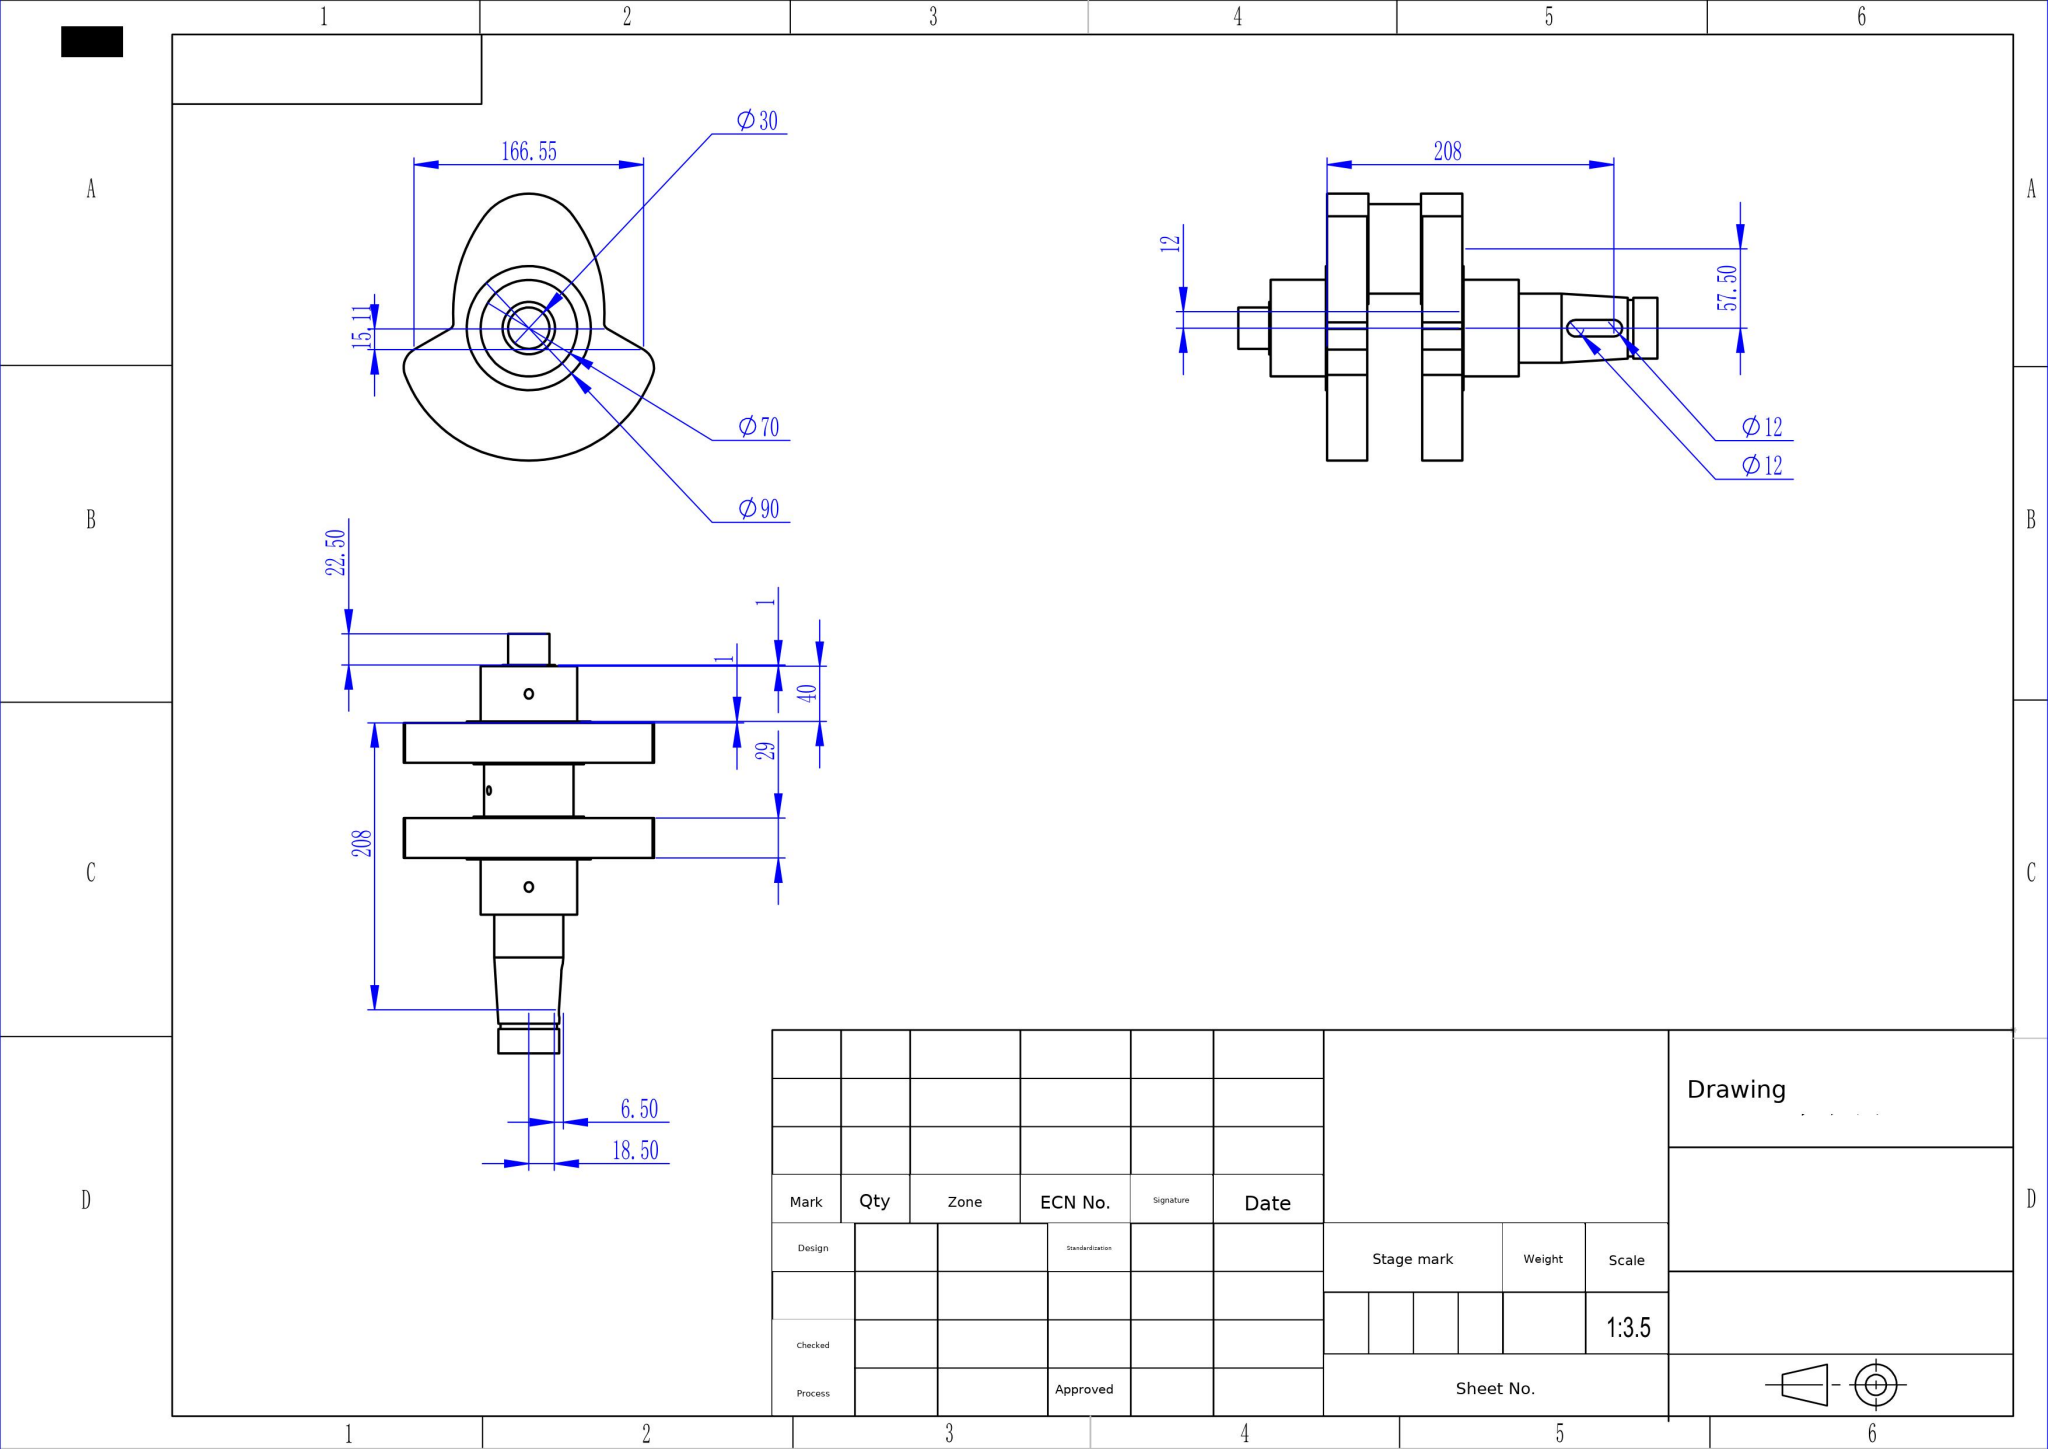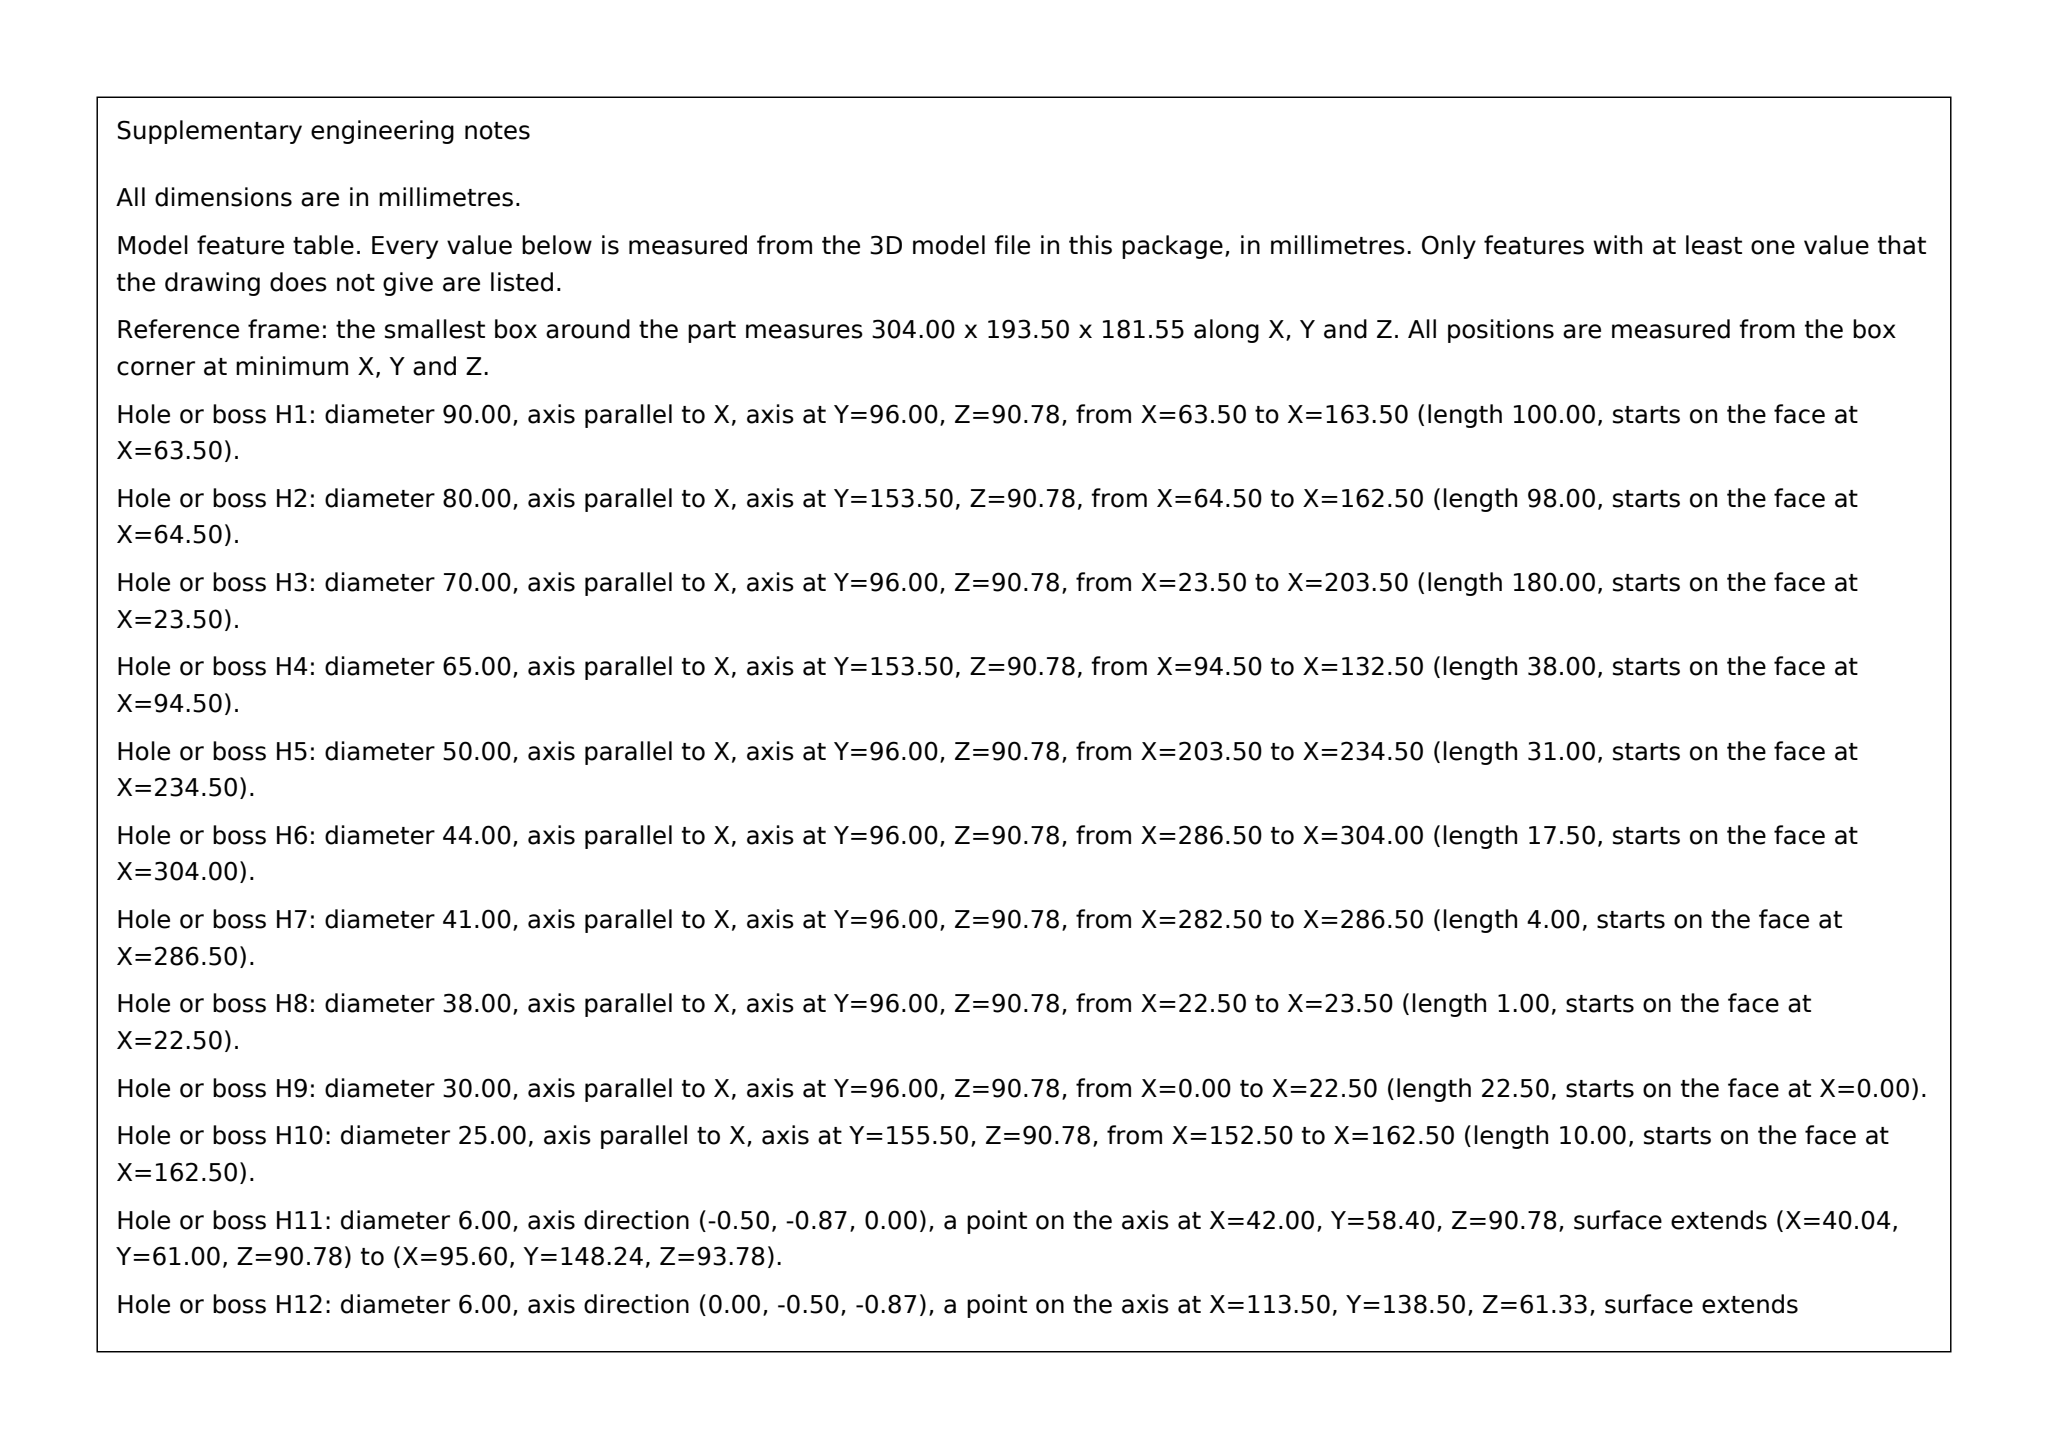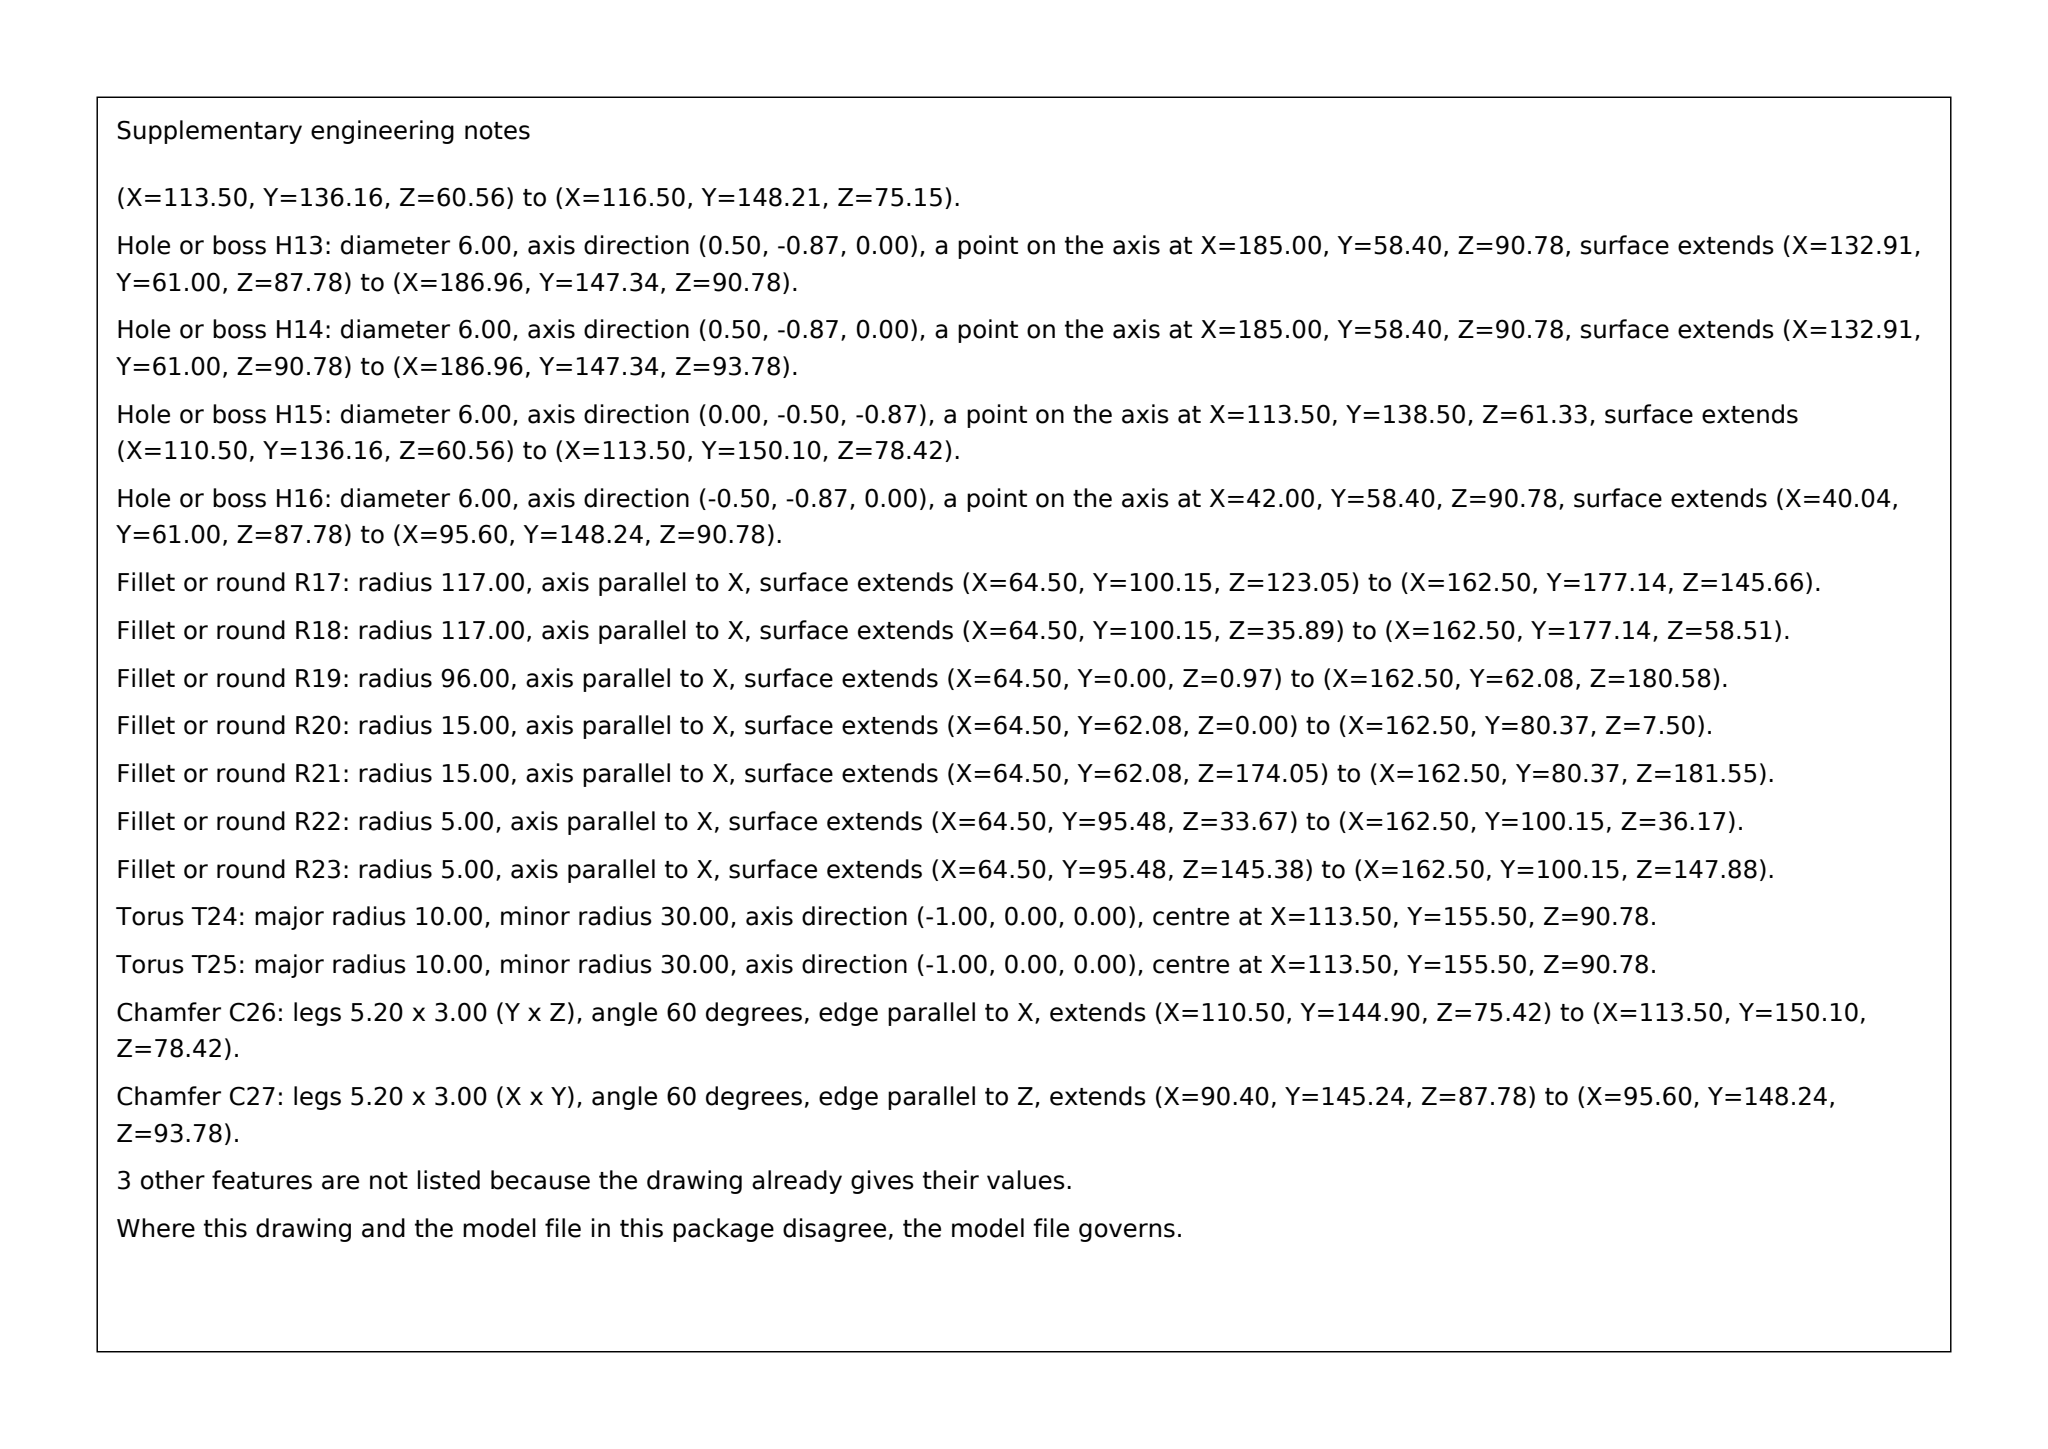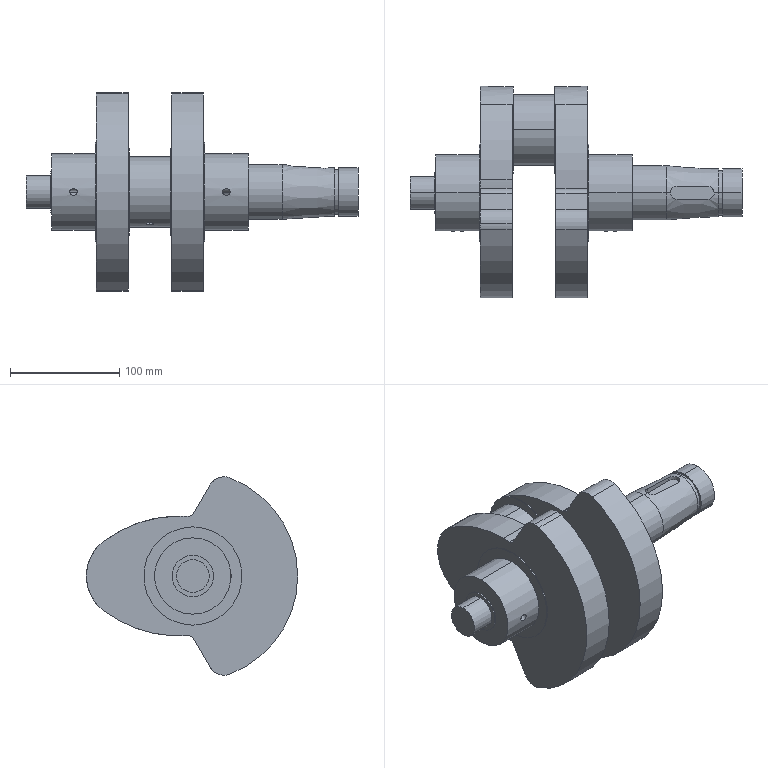Part | SolidWorks | mm | 1 solid | 86 faces | box 304 x 193.5 x 181.55 mm | volume 1902871 mm3 | cylinder 55 | plane 27 | torus 2 | cone 2 | commonest cylinder face diameters 30 x8 6 x6 234 x6 10 x6 70 x4 90 x4 80 x4 12 x3